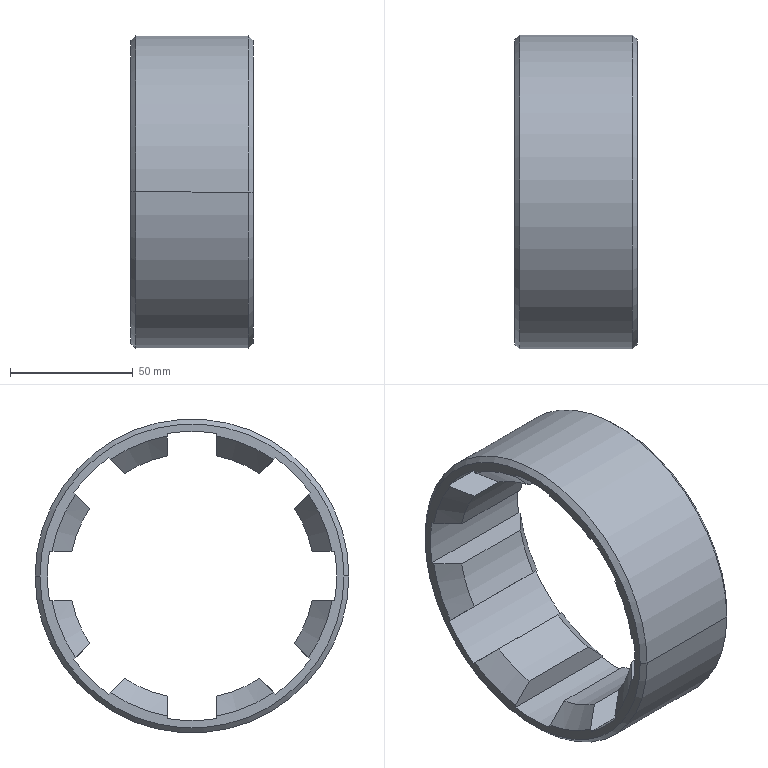Component | SolidWorks | 216OuterTube-1_CenteringRing-1 | 1 solid | 57 faces | box 50 x 128 x 128 mm | volume 165818 mm3 | cone 20 | cylinder 19 | plane 18 | commonest cylinder face diameters 118 x9 100 x8 128 x2 | material Brass
build123d program:
from build123d import *

# Parameters (mm, degrees)
CUT_EXTRUDE1_DEPTH = 104.402
CIRPATTERN1_COUNT  = 8


with BuildPart() as part:
    # Model → Revolve1 (revolve)
    with BuildSketch(Plane.XY):
        Polygon((8, 50), (42, 50), (50, 58), (50, 62), (48, 64), (2, 64), (0, 62), (0, 58), align=None)
    revolve(axis=Axis((36.145, 0, 0), (-1, 0, 0)))

    # Sketch2 → Cut-Extrude1 (cut, through all)
    with BuildSketch(Plane.ZY):
        with BuildLine():
            Line((-10, 58.146), (-10, 46.435))
            ThreePointArc((-10, 46.435), (0, 47.5), (10, 46.435))
            Line((10, 46.435), (10, 58.146))
            ThreePointArc((10, 58.146), (0, 59), (-10, 58.146))
        make_face()
    cut_extrude1 = extrude(amount=-CUT_EXTRUDE1_DEPTH, mode=Mode.SUBTRACT)

    # CirPattern1: Cut-Extrude1 ×8 about axis
    cirpattern1_axis = Axis((0, 0, 0), (1, 0, 0))
    for i in range(1, CIRPATTERN1_COUNT):
        add(cut_extrude1.rotate(cirpattern1_axis, i * 360 / CIRPATTERN1_COUNT), mode=Mode.SUBTRACT)


solid = part.part

# Placed as in the assembly
solid = solid.moved(Location((2555.079, 0, 0), (0, 0, 0)))